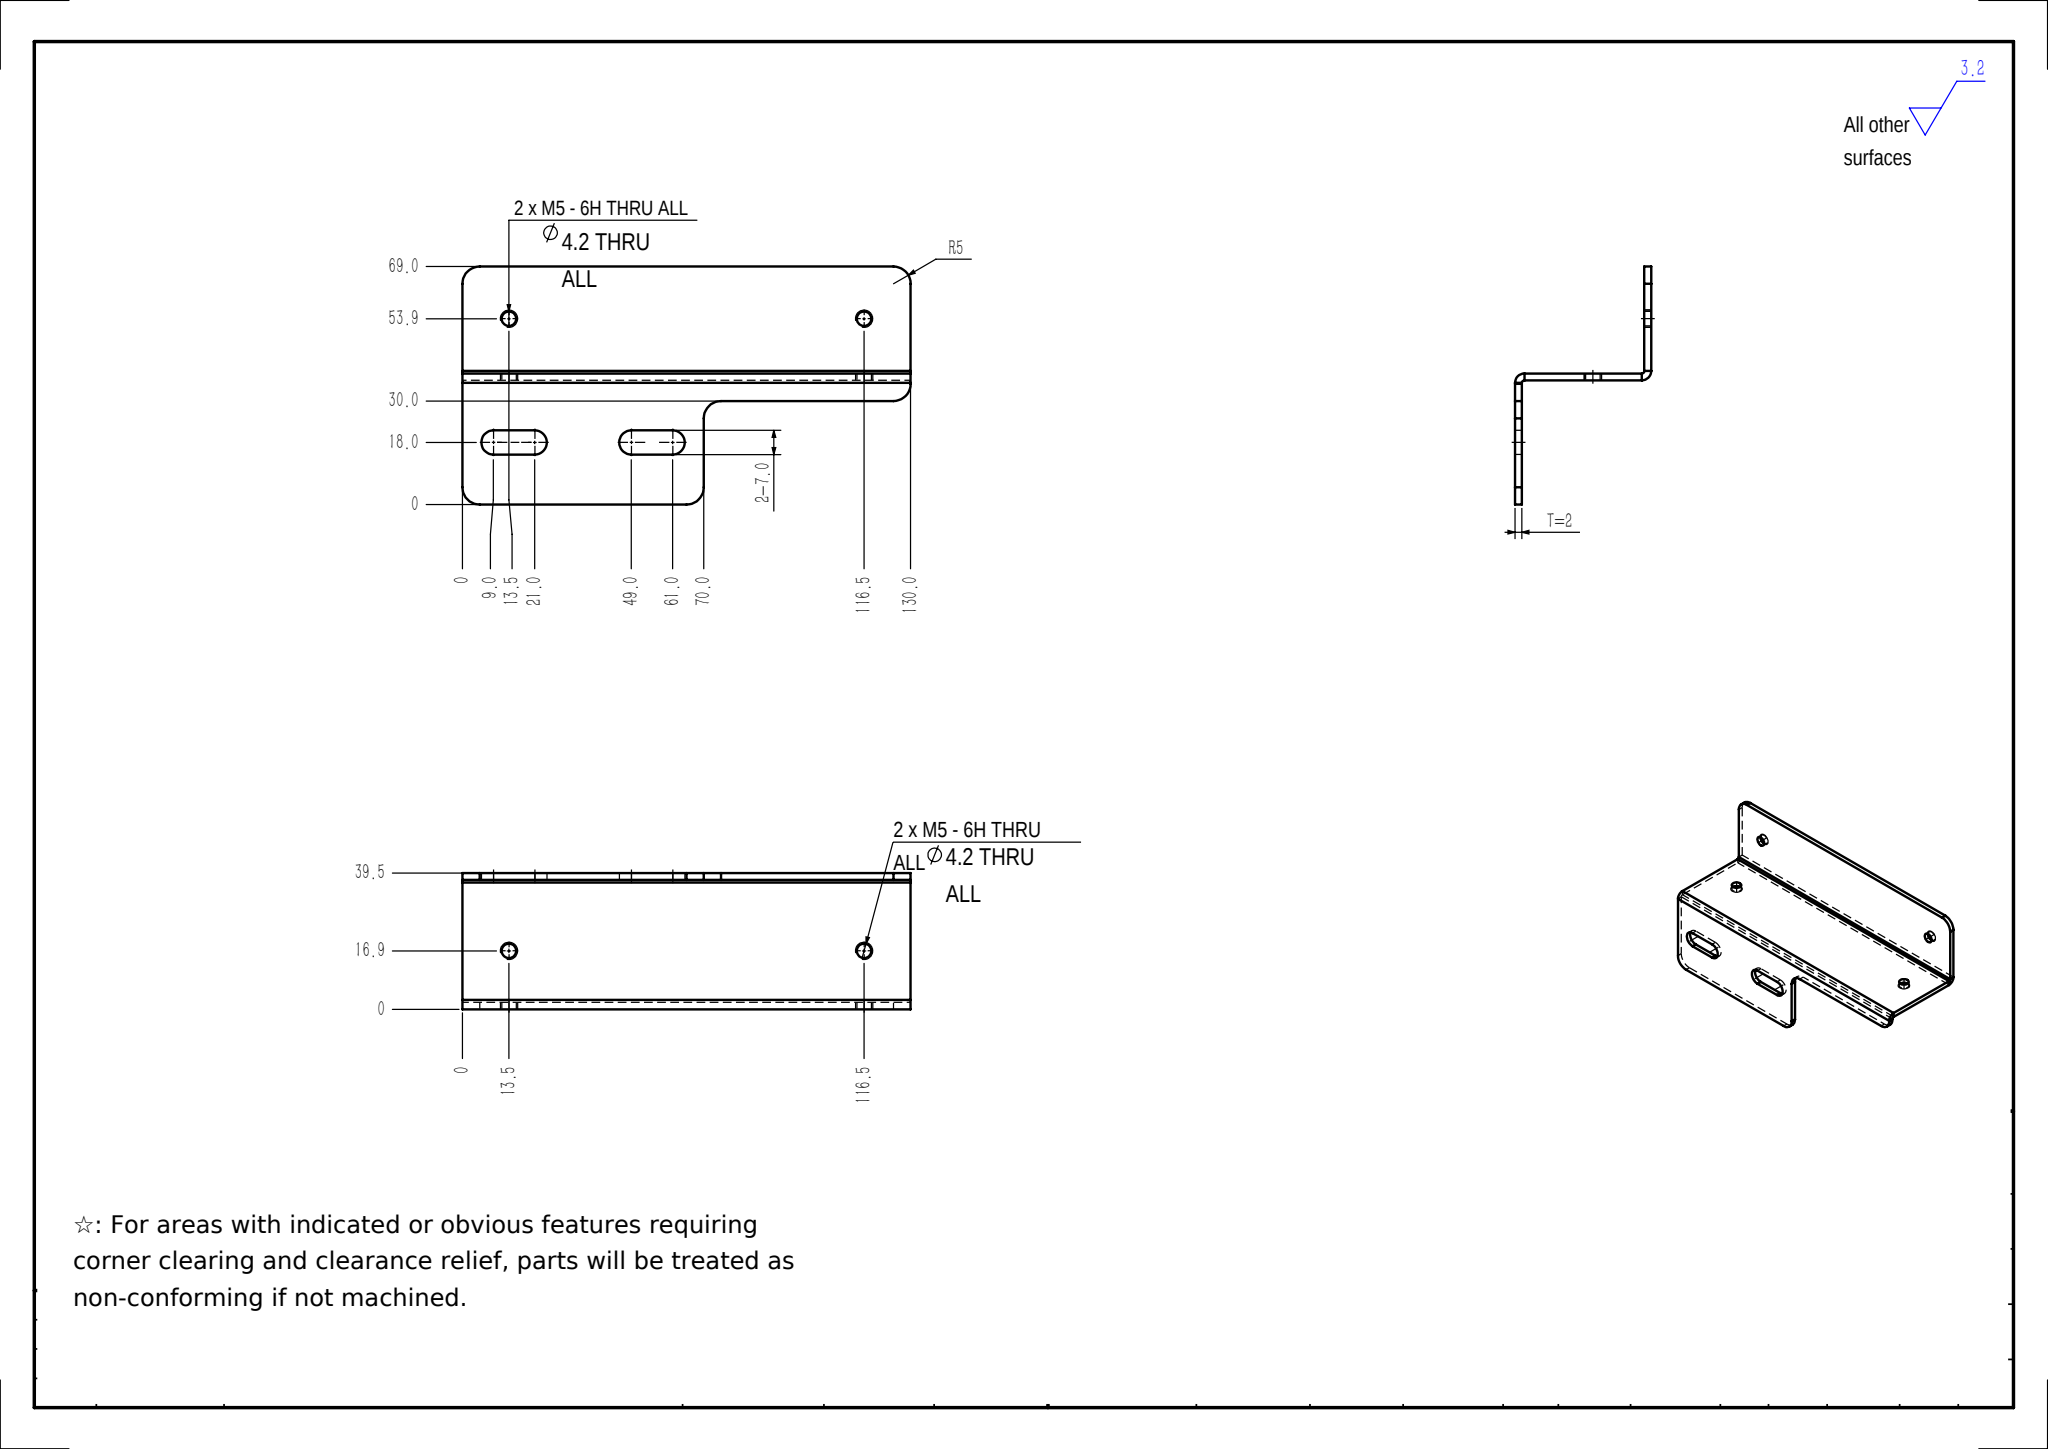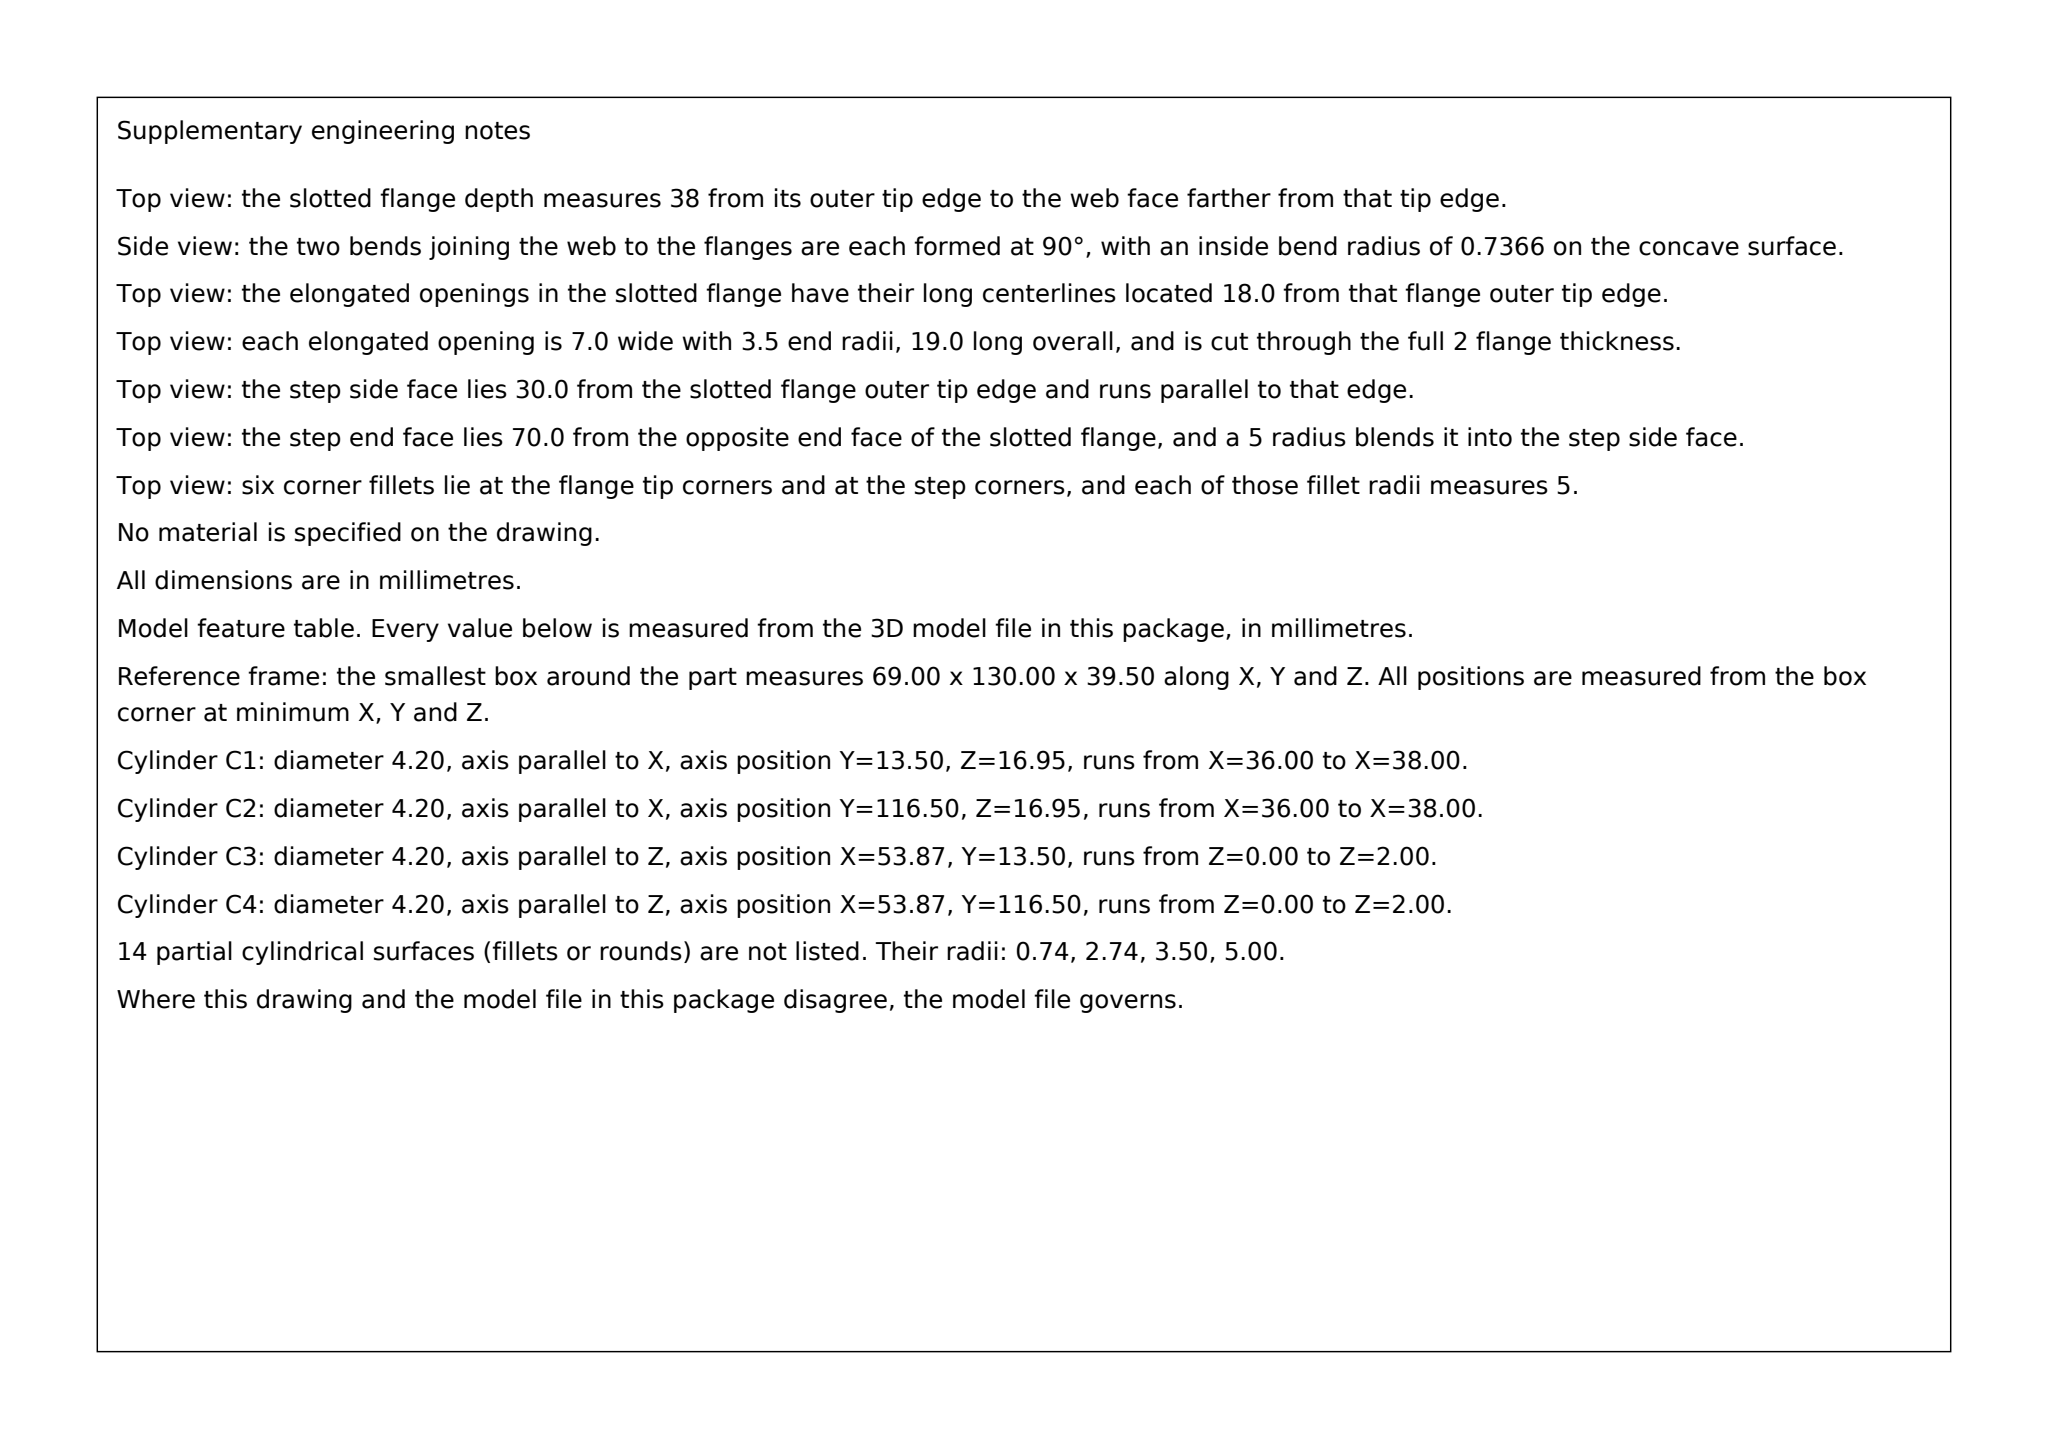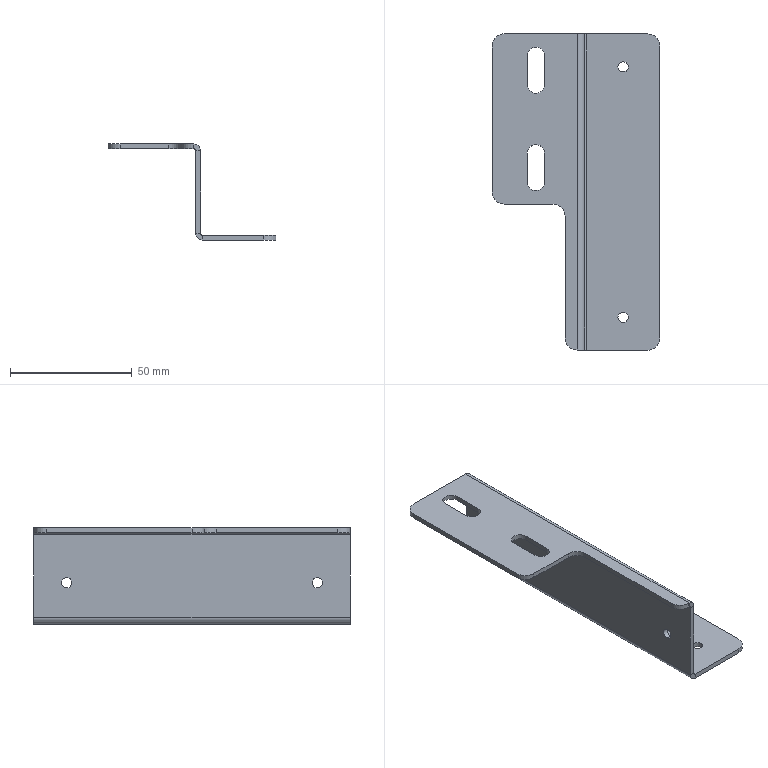Part | SolidWorks | mm | 1 solid | 46 faces | box 69 x 130 x 39.5 mm | volume 23059 mm3 | plane 24 | cylinder 22 | commonest cylinder face diameters 4.2 x8 10 x6 7 x4 5.473 x2 1.473 x2
Drawing notes:
ALL BENDS R0.74 INR / R2.74 OUTR, T=2 | from the solid: Cylinders dia 1.473 & 5.473 abt Y axis at (35.26,36.76) and (38.74,2.74), L=130 -> R0.737 inner, R2.737 outer with T=2
BEND LINES AT 36.0 & 38.0 FROM 0 (69 DIR); FLGS 38 & 31 WIDE | from the solid: X-normal planes at 0, 36.0, 38.0, 69.0; web 2 thk between x=36 and x=38; bottom flg x=0-38, top flg x=38-69
ALL CORNER & NOTCH FILLETS R5 TYP | from the solid: Z-axis cylinders dia 10.0 at (5,65),(5,125),(25,55),(35,5),(64,5),(64,125), L=2 -> R5